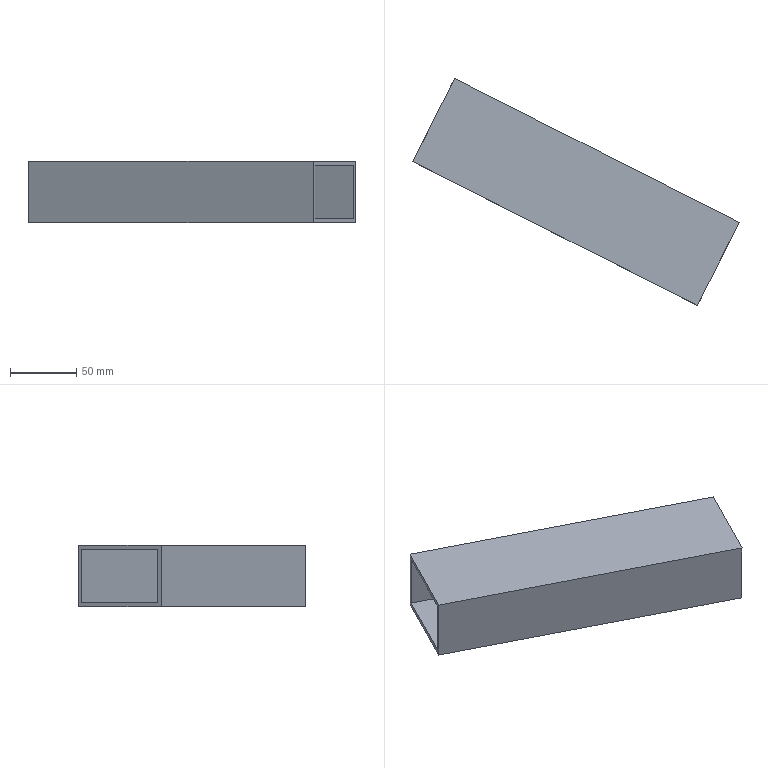Component | SolidWorks | FrameAssemblyDrawing11111-1_Part5-1 | 1 solid | 10 faces | box 245.72 x 170.94 x 46 mm | volume 158400 mm3 | plane 10
build123d program:
from build123d import *

# Parameters (mm, degrees)
SKETCH1_W           = 240
SKETCH1_H           = 70
BOSS_EXTRUDE1_DEPTH = 46
SHELL10_T           = -3


with BuildPart() as part:
    # Sketch1 → Boss-Extrude1 (new body)
    with BuildSketch(Plane.XY):
        with Locations((58.859, 46.187)):
            Rectangle(SKETCH1_W, SKETCH1_H)
    extrude(amount=BOSS_EXTRUDE1_DEPTH)

    # Shell10
    shell10_openings = [part.faces().sort_by_distance(p)[0] for p in [
        (178.859, 46.187, 23),
        (-61.141, 46.187, 23),
    ]]
    offset(amount=SHELL10_T, openings=shell10_openings, kind=Kind.INTERSECTION)


solid = part.part

# Placed as in the assembly
solid = solid.moved(Location((-1495.399, -380.35, 1040.971), (0, 0, -26.879)))
STEP:
#1=COLOUR_RGB('',0.7922,0.8196,0.9333);
#2=FILL_AREA_STYLE_COLOUR('',#1);
#3=FILL_AREA_STYLE('',(#2));
#4=SURFACE_STYLE_FILL_AREA(#3);
#5=SURFACE_SIDE_STYLE('',(#4));
#6=SURFACE_STYLE_USAGE(.BOTH.,#5);
#7=PRESENTATION_STYLE_ASSIGNMENT((#6));
#8=CARTESIAN_POINT('',(-59.576,-11.035,40.983));
#9=VERTEX_POINT('',#8);
#10=CARTESIAN_POINT('',(-60.822,-13.493,40.983));
#11=VERTEX_POINT('',#10);
#12=CARTESIAN_POINT('',(-60.822,-13.493,40.983));
#13=DIRECTION('',(-0.4521,-0.892,-0.));
#14=VECTOR('',#13,39.37);
#15=LINE('',#12,#14);
#16=EDGE_CURVE('',#9,#11,#15,.T.);
#17=ORIENTED_EDGE('',*,*,#16,.T.);
#18=CARTESIAN_POINT('',(-60.822,-13.493,42.794));
#19=VERTEX_POINT('',#18);
#20=CARTESIAN_POINT('',(-60.822,-13.493,42.794));
#21=DIRECTION('',(0.,0.,-1.));
#22=VECTOR('',#21,39.37);
#23=LINE('',#20,#22);
#24=EDGE_CURVE('',#19,#11,#23,.T.);
#25=ORIENTED_EDGE('',*,*,#24,.F.);
#26=CARTESIAN_POINT('',(-59.576,-11.035,42.794));
#27=VERTEX_POINT('',#26);
#28=CARTESIAN_POINT('',(-60.822,-13.493,42.794));
#29=DIRECTION('',(-0.4521,-0.892,-0.));
#30=VECTOR('',#29,39.37);
#31=LINE('',#28,#30);
#32=EDGE_CURVE('',#27,#19,#31,.T.);
#33=ORIENTED_EDGE('',*,*,#32,.F.);
#34=CARTESIAN_POINT('',(-59.576,-11.035,42.794));
#35=DIRECTION('',(0.,0.,-1.));
#36=VECTOR('',#35,39.37);
#37=LINE('',#34,#36);
#38=EDGE_CURVE('',#27,#9,#37,.T.);
#39=ORIENTED_EDGE('',*,*,#38,.T.);
#40=EDGE_LOOP('',(#17,#25,#33,#39));
#41=FACE_OUTER_BOUND('',#40,.T.);
#42=CARTESIAN_POINT('',(-59.629,-11.14,41.101));
#43=VERTEX_POINT('',#42);
#44=CARTESIAN_POINT('',(-60.769,-13.388,41.101));
#45=VERTEX_POINT('',#44);
#46=CARTESIAN_POINT('',(-61.021,-13.886,41.101));
#47=DIRECTION('',(-0.4521,-0.892,-0.));
#48=VECTOR('',#47,39.37);
#49=LINE('',#46,#48);
#50=EDGE_CURVE('',#43,#45,#49,.T.);
#51=ORIENTED_EDGE('',*,*,#50,.F.);
#52=CARTESIAN_POINT('',(-59.629,-11.14,42.676));
#53=VERTEX_POINT('',#52);
#54=CARTESIAN_POINT('',(-59.629,-11.14,42.794));
#55=DIRECTION('',(0.,0.,-1.));
#56=VECTOR('',#55,39.37);
#57=LINE('',#54,#56);
#58=EDGE_CURVE('',#53,#43,#57,.T.);
#59=ORIENTED_EDGE('',*,*,#58,.F.);
#60=CARTESIAN_POINT('',(-60.769,-13.388,42.676));
#61=VERTEX_POINT('',#60);
#62=CARTESIAN_POINT('',(-61.021,-13.886,42.676));
#63=DIRECTION('',(-0.4521,-0.892,-0.));
#64=VECTOR('',#63,39.37);
#65=LINE('',#62,#64);
#66=EDGE_CURVE('',#53,#61,#65,.T.);
#67=ORIENTED_EDGE('',*,*,#66,.T.);
#68=CARTESIAN_POINT('',(-60.769,-13.388,42.794));
#69=DIRECTION('',(0.,0.,-1.));
#70=VECTOR('',#69,39.37);
#71=LINE('',#68,#70);
#72=EDGE_CURVE('',#61,#45,#71,.T.);
#73=ORIENTED_EDGE('',*,*,#72,.T.);
#74=EDGE_LOOP('',(#51,#59,#67,#73));
#75=FACE_BOUND('',#74,.T.);
#76=CARTESIAN_POINT('',(-60.822,-13.493,42.794));
#77=DIRECTION('',(0.892,-0.4521,-0.));
#78=DIRECTION('',(0.,0.,-1.));
#79=AXIS2_PLACEMENT_3D('',#76,#77,#78);
#80=PLANE('',#79);
#81=ADVANCED_FACE('',(#41,#75),#80,.F.);
#82=CARTESIAN_POINT('',(-52.394,-17.765,40.983));
#83=VERTEX_POINT('',#82);
#84=CARTESIAN_POINT('',(-51.148,-15.307,40.983));
#85=VERTEX_POINT('',#84);
#86=CARTESIAN_POINT('',(-51.148,-15.307,40.983));
#87=DIRECTION('',(0.4521,0.892,0.));
#88=VECTOR('',#87,39.37);
#89=LINE('',#86,#88);
#90=EDGE_CURVE('',#83,#85,#89,.T.);
#91=ORIENTED_EDGE('',*,*,#90,.T.);
#92=CARTESIAN_POINT('',(-51.148,-15.307,42.794));
#93=VERTEX_POINT('',#92);
#94=CARTESIAN_POINT('',(-51.148,-15.307,42.794));
#95=DIRECTION('',(0.,0.,-1.));
#96=VECTOR('',#95,39.37);
#97=LINE('',#94,#96);
#98=EDGE_CURVE('',#93,#85,#97,.T.);
#99=ORIENTED_EDGE('',*,*,#98,.F.);
#100=CARTESIAN_POINT('',(-52.394,-17.765,42.794));
#101=VERTEX_POINT('',#100);
#102=CARTESIAN_POINT('',(-51.148,-15.307,42.794));
#103=DIRECTION('',(0.4521,0.892,0.));
#104=VECTOR('',#103,39.37);
#105=LINE('',#102,#104);
#106=EDGE_CURVE('',#101,#93,#105,.T.);
#107=ORIENTED_EDGE('',*,*,#106,.F.);
#108=CARTESIAN_POINT('',(-52.394,-17.765,42.794));
#109=DIRECTION('',(0.,0.,-1.));
#110=VECTOR('',#109,39.37);
#111=LINE('',#108,#110);
#112=EDGE_CURVE('',#101,#83,#111,.T.);
#113=ORIENTED_EDGE('',*,*,#112,.T.);
#114=EDGE_LOOP('',(#91,#99,#107,#113));
#115=FACE_OUTER_BOUND('',#114,.T.);
#116=CARTESIAN_POINT('',(-52.341,-17.66,41.101));
#117=VERTEX_POINT('',#116);
#118=CARTESIAN_POINT('',(-51.201,-15.412,41.101));
#119=VERTEX_POINT('',#118);
#120=CARTESIAN_POINT('',(-52.593,-18.158,41.101));
#121=DIRECTION('',(0.4521,0.892,0.));
#122=VECTOR('',#121,39.37);
#123=LINE('',#120,#122);
#124=EDGE_CURVE('',#117,#119,#123,.T.);
#125=ORIENTED_EDGE('',*,*,#124,.F.);
#126=CARTESIAN_POINT('',(-52.341,-17.66,42.676));
#127=VERTEX_POINT('',#126);
#128=CARTESIAN_POINT('',(-52.341,-17.66,42.794));
#129=DIRECTION('',(0.,0.,-1.));
#130=VECTOR('',#129,39.37);
#131=LINE('',#128,#130);
#132=EDGE_CURVE('',#127,#117,#131,.T.);
#133=ORIENTED_EDGE('',*,*,#132,.F.);
#134=CARTESIAN_POINT('',(-51.201,-15.412,42.676));
#135=VERTEX_POINT('',#134);
#136=CARTESIAN_POINT('',(-52.593,-18.158,42.676));
#137=DIRECTION('',(0.4521,0.892,0.));
#138=VECTOR('',#137,39.37);
#139=LINE('',#136,#138);
#140=EDGE_CURVE('',#127,#135,#139,.T.);
#141=ORIENTED_EDGE('',*,*,#140,.T.);
#142=CARTESIAN_POINT('',(-51.201,-15.412,42.794));
#143=DIRECTION('',(0.,0.,-1.));
#144=VECTOR('',#143,39.37);
#145=LINE('',#142,#144);
#146=EDGE_CURVE('',#135,#119,#145,.T.);
#147=ORIENTED_EDGE('',*,*,#146,.T.);
#148=EDGE_LOOP('',(#125,#133,#141,#147));
#149=FACE_BOUND('',#148,.T.);
#150=CARTESIAN_POINT('',(-51.148,-15.307,42.794));
#151=DIRECTION('',(-0.892,0.4521,0.));
#152=DIRECTION('',(-0.,-0.,1.));
#153=AXIS2_PLACEMENT_3D('',#150,#151,#152);
#154=PLANE('',#153);
#155=ADVANCED_FACE('',(#115,#149),#154,.F.);
#156=CARTESIAN_POINT('',(-60.822,-13.493,40.983));
#157=DIRECTION('',(0.892,-0.4521,-0.));
#158=VECTOR('',#157,39.37);
#159=LINE('',#156,#158);
#160=EDGE_CURVE('',#11,#83,#159,.T.);
#161=ORIENTED_EDGE('',*,*,#160,.T.);
#162=ORIENTED_EDGE('',*,*,#112,.F.);
#163=CARTESIAN_POINT('',(-60.822,-13.493,42.794));
#164=DIRECTION('',(0.892,-0.4521,-0.));
#165=VECTOR('',#164,39.37);
#166=LINE('',#163,#165);
#167=EDGE_CURVE('',#19,#101,#166,.T.);
#168=ORIENTED_EDGE('',*,*,#167,.F.);
#169=ORIENTED_EDGE('',*,*,#24,.T.);
#170=EDGE_LOOP('',(#161,#162,#168,#169));
#171=FACE_OUTER_BOUND('',#170,.T.);
#172=CARTESIAN_POINT('',(-60.822,-13.493,42.794));
#173=DIRECTION('',(0.4521,0.892,0.));
#174=DIRECTION('',(-0.,-0.,1.));
#175=AXIS2_PLACEMENT_3D('',#172,#173,#174);
#176=PLANE('',#175);
#177=ADVANCED_FACE('',(#171),#176,.F.);
#178=CARTESIAN_POINT('',(-59.576,-11.035,40.983));
#179=DIRECTION('',(-0.892,0.4521,0.));
#180=VECTOR('',#179,39.37);
#181=LINE('',#178,#180);
#182=EDGE_CURVE('',#85,#9,#181,.T.);
#183=ORIENTED_EDGE('',*,*,#182,.T.);
#184=ORIENTED_EDGE('',*,*,#38,.F.);
#185=CARTESIAN_POINT('',(-59.576,-11.035,42.794));
#186=DIRECTION('',(-0.892,0.4521,0.));
#187=VECTOR('',#186,39.37);
#188=LINE('',#185,#187);
#189=EDGE_CURVE('',#93,#27,#188,.T.);
#190=ORIENTED_EDGE('',*,*,#189,.F.);
#191=ORIENTED_EDGE('',*,*,#98,.T.);
#192=EDGE_LOOP('',(#183,#184,#190,#191));
#193=FACE_OUTER_BOUND('',#192,.T.);
#194=CARTESIAN_POINT('',(-59.576,-11.035,42.794));
#195=DIRECTION('',(-0.4521,-0.892,-0.));
#196=DIRECTION('',(0.,0.,-1.));
#197=AXIS2_PLACEMENT_3D('',#194,#195,#196);
#198=PLANE('',#197);
#199=ADVANCED_FACE('',(#193),#198,.F.);
#200=ORIENTED_EDGE('',*,*,#32,.T.);
#201=ORIENTED_EDGE('',*,*,#167,.T.);
#202=ORIENTED_EDGE('',*,*,#106,.T.);
#203=ORIENTED_EDGE('',*,*,#189,.T.);
#204=EDGE_LOOP('',(#200,#201,#202,#203));
#205=FACE_OUTER_BOUND('',#204,.T.);
#206=CARTESIAN_POINT('',(-58.874,-14.974,42.794));
#207=DIRECTION('',(0.,0.,-1.));
#208=DIRECTION('',(-0.892,0.4521,0.));
#209=AXIS2_PLACEMENT_3D('',#206,#207,#208);
#210=PLANE('',#209);
#211=ADVANCED_FACE('',(#205),#210,.F.);
#212=ORIENTED_EDGE('',*,*,#16,.F.);
#213=ORIENTED_EDGE('',*,*,#182,.F.);
#214=ORIENTED_EDGE('',*,*,#90,.F.);
#215=ORIENTED_EDGE('',*,*,#160,.F.);
#216=EDGE_LOOP('',(#212,#213,#214,#215));
#217=FACE_OUTER_BOUND('',#216,.T.);
#218=CARTESIAN_POINT('',(-58.874,-14.974,40.983));
#219=DIRECTION('',(0.,0.,-1.));
#220=DIRECTION('',(-0.892,0.4521,0.));
#221=AXIS2_PLACEMENT_3D('',#218,#219,#220);
#222=PLANE('',#221);
#223=ADVANCED_FACE('',(#217),#222,.T.);
#224=CARTESIAN_POINT('',(-58.621,-14.476,41.101));
#225=DIRECTION('',(0.892,-0.4521,-0.));
#226=VECTOR('',#225,39.37);
#227=LINE('',#224,#226);
#228=EDGE_CURVE('',#45,#117,#227,.T.);
#229=ORIENTED_EDGE('',*,*,#228,.F.);
#230=ORIENTED_EDGE('',*,*,#72,.F.);
#231=CARTESIAN_POINT('',(-58.621,-14.476,42.676));
#232=DIRECTION('',(0.892,-0.4521,-0.));
#233=VECTOR('',#232,39.37);
#234=LINE('',#231,#233);
#235=EDGE_CURVE('',#61,#127,#234,.T.);
#236=ORIENTED_EDGE('',*,*,#235,.T.);
#237=ORIENTED_EDGE('',*,*,#132,.T.);
#238=EDGE_LOOP('',(#229,#230,#236,#237));
#239=FACE_OUTER_BOUND('',#238,.T.);
#240=CARTESIAN_POINT('',(-60.769,-13.388,42.794));
#241=DIRECTION('',(0.4521,0.892,0.));
#242=DIRECTION('',(-0.,-0.,1.));
#243=AXIS2_PLACEMENT_3D('',#240,#241,#242);
#244=PLANE('',#243);
#245=ADVANCED_FACE('',(#239),#244,.T.);
#246=CARTESIAN_POINT('',(-57.482,-12.229,41.101));
#247=DIRECTION('',(-0.892,0.4521,0.));
#248=VECTOR('',#247,39.37);
#249=LINE('',#246,#248);
#250=EDGE_CURVE('',#119,#43,#249,.T.);
#251=ORIENTED_EDGE('',*,*,#250,.F.);
#252=ORIENTED_EDGE('',*,*,#146,.F.);
#253=CARTESIAN_POINT('',(-57.482,-12.229,42.676));
#254=DIRECTION('',(-0.892,0.4521,0.));
#255=VECTOR('',#254,39.37);
#256=LINE('',#253,#255);
#257=EDGE_CURVE('',#135,#53,#256,.T.);
#258=ORIENTED_EDGE('',*,*,#257,.T.);
#259=ORIENTED_EDGE('',*,*,#58,.T.);
#260=EDGE_LOOP('',(#251,#252,#258,#259));
#261=FACE_OUTER_BOUND('',#260,.T.);
#262=CARTESIAN_POINT('',(-59.629,-11.14,42.794));
#263=DIRECTION('',(-0.4521,-0.892,-0.));
#264=DIRECTION('',(0.,0.,-1.));
#265=AXIS2_PLACEMENT_3D('',#262,#263,#264);
#266=PLANE('',#265);
#267=ADVANCED_FACE('',(#261),#266,.T.);
#268=ORIENTED_EDGE('',*,*,#66,.F.);
#269=ORIENTED_EDGE('',*,*,#257,.F.);
#270=ORIENTED_EDGE('',*,*,#140,.F.);
#271=ORIENTED_EDGE('',*,*,#235,.F.);
#272=EDGE_LOOP('',(#268,#269,#270,#271));
#273=FACE_OUTER_BOUND('',#272,.T.);
#274=CARTESIAN_POINT('',(-58.874,-14.974,42.676));
#275=DIRECTION('',(0.,0.,-1.));
#276=DIRECTION('',(-0.892,0.4521,0.));
#277=AXIS2_PLACEMENT_3D('',#274,#275,#276);
#278=PLANE('',#277);
#279=ADVANCED_FACE('',(#273),#278,.T.);
#280=ORIENTED_EDGE('',*,*,#50,.T.);
#281=ORIENTED_EDGE('',*,*,#228,.T.);
#282=ORIENTED_EDGE('',*,*,#124,.T.);
#283=ORIENTED_EDGE('',*,*,#250,.T.);
#284=EDGE_LOOP('',(#280,#281,#282,#283));
#285=FACE_OUTER_BOUND('',#284,.T.);
#286=CARTESIAN_POINT('',(-58.874,-14.974,41.101));
#287=DIRECTION('',(0.,0.,-1.));
#288=DIRECTION('',(-0.892,0.4521,0.));
#289=AXIS2_PLACEMENT_3D('',#286,#287,#288);
#290=PLANE('',#289);
#291=ADVANCED_FACE('',(#285),#290,.F.);
#292=CLOSED_SHELL('',(#81,#155,#177,#199,#211,#223,#245,#267,#279,#291));
#293=MANIFOLD_SOLID_BREP('',#292);
#294=STYLED_ITEM('',(#7),#293);
#295=PRESENTATION_LAYER_ASSIGNMENT('','',(#294));
#296=(LENGTH_UNIT()NAMED_UNIT(*)SI_UNIT($,.METRE.));
#297=LENGTH_MEASURE_WITH_UNIT(LENGTH_MEASURE(0.0254),#296);
#298=DIMENSIONAL_EXPONENTS(1.,0.,0.,0.,0.,0.,0.);
#299=(CONVERSION_BASED_UNIT('',#297)LENGTH_UNIT()NAMED_UNIT(#298));
#300=UNCERTAINTY_MEASURE_WITH_UNIT(LENGTH_MEASURE(0.00001),#299,'','');
#301=(NAMED_UNIT(*)PLANE_ANGLE_UNIT()SI_UNIT($,.RADIAN.));
#302=(NAMED_UNIT(*)SI_UNIT($,.STERADIAN.)SOLID_ANGLE_UNIT());
#303=(GEOMETRIC_REPRESENTATION_CONTEXT(3)GLOBAL_UNCERTAINTY_ASSIGNED_CONTEXT((#300))GLOBAL_UNIT_ASSIGNED_CONTEXT((#299,#301,#302))REPRESENTATION_CONTEXT('',''));
#304=MECHANICAL_DESIGN_GEOMETRIC_PRESENTATION_REPRESENTATION('',(#294),#303);
#305=CARTESIAN_POINT('',(0.,0.,0.));
#306=DIRECTION('',(0.,0.,1.));
#307=DIRECTION('',(1.,0.,0.));
#308=AXIS2_PLACEMENT_3D('',#305,#306,#307);
#309=(LENGTH_UNIT()NAMED_UNIT(*)SI_UNIT($,.METRE.));
#310=LENGTH_MEASURE_WITH_UNIT(LENGTH_MEASURE(0.0254),#309);
#311=DIMENSIONAL_EXPONENTS(1.,0.,0.,0.,0.,0.,0.);
#312=(CONVERSION_BASED_UNIT('',#310)LENGTH_UNIT()NAMED_UNIT(#311));
#313=UNCERTAINTY_MEASURE_WITH_UNIT(LENGTH_MEASURE(0.00001),#312,'','');
#314=(NAMED_UNIT(*)PLANE_ANGLE_UNIT()SI_UNIT($,.RADIAN.));
#315=(NAMED_UNIT(*)SI_UNIT($,.STERADIAN.)SOLID_ANGLE_UNIT());
#316=(GEOMETRIC_REPRESENTATION_CONTEXT(3)GLOBAL_UNCERTAINTY_ASSIGNED_CONTEXT((#313))GLOBAL_UNIT_ASSIGNED_CONTEXT((#312,#314,#315))REPRESENTATION_CONTEXT('',''));
#317=ADVANCED_BREP_SHAPE_REPRESENTATION('',(#293,#308),#316);